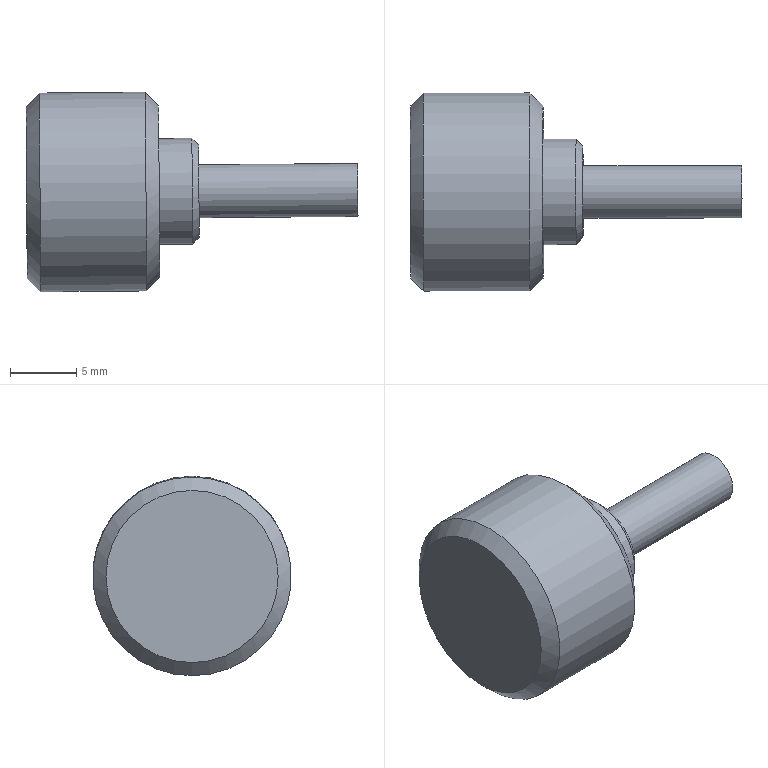Component | NX | INDICATOR_LOCK_HANDWHEEL | 1 solid | 10 faces | box 25.06 x 15.01 x 15.06 mm | volume 2021 mm3 | plane 4 | cylinder 3 | cone 3 | commonest cylinder face diameters 4 x1 8 x1 15 x1
STEP:
#1=CARTESIAN_POINT('',(0.,0.,0.));
#2=DIRECTION('',(0.,0.,1.));
#3=DIRECTION('',(1.,0.,0.));
#4=AXIS2_PLACEMENT_3D('',#1,#2,#3);
#5=CARTESIAN_POINT('',(65.216,280.465,124.861));
#6=VERTEX_POINT('',#5);
#7=CARTESIAN_POINT('',(65.167,280.465,131.36));
#8=DIRECTION('',(-1.,-0.001327,-0.007524));
#9=DIRECTION('',(0.007524,0.00000499,-1.));
#10=AXIS2_PLACEMENT_3D('',#7,#8,#9);
#11=CIRCLE('',#10,6.5);
#12=CARTESIAN_POINT('',(65.11,280.465,138.86));
#13=DIRECTION('',(1.,0.001327,0.007524));
#14=DIRECTION('',(0.007524,0.00000499,-1.));
#15=AXIS2_PLACEMENT_3D('',#12,#13,#14);
#16=PLANE('',#15);
#17=CARTESIAN_POINT('',(14.,-0.));
#18=CARTESIAN_POINT('',(14.,-11.258));
#19=CARTESIAN_POINT('',(4.25,-5.629));
#20=CARTESIAN_POINT('',(-5.5,-0.));
#21=CARTESIAN_POINT('',(4.25,5.629));
#22=CARTESIAN_POINT('',(14.,11.258));
#23=CARTESIAN_POINT('',(14.,-0.));
#24=(BOUNDED_CURVE()B_SPLINE_CURVE(2,(#17,#18,#19,#20,#21,#22,#23),.UNSPECIFIED.,.T.,.F.)B_SPLINE_CURVE_WITH_KNOTS((1,2,2,2,2,1),(-2.094,0.,2.094,4.189,6.283,8.378),.UNSPECIFIED.)CURVE()GEOMETRIC_REPRESENTATION_ITEM()RATIONAL_B_SPLINE_CURVE((1.,0.5,1.,0.5,1.,0.5,1.))REPRESENTATION_ITEM(''));
#25=(GEOMETRIC_REPRESENTATION_CONTEXT(2)PARAMETRIC_REPRESENTATION_CONTEXT()REPRESENTATION_CONTEXT('',''));
#26=DEFINITIONAL_REPRESENTATION('',(#24),#25);
#27=PCURVE('',#16,#26);
#28=CARTESIAN_POINT('',(65.167,280.465,131.36));
#29=DIRECTION('',(1.,0.001327,0.007524));
#30=DIRECTION('',(0.007524,0.00000499,-1.));
#31=AXIS2_PLACEMENT_3D('',#28,#29,#30);
#32=CONICAL_SURFACE('',#31,6.5,0.7854);
#33=CARTESIAN_POINT('',(6.283,0.));
#34=DIRECTION('',(-1.,0.));
#35=VECTOR('',#34,1.);
#36=LINE('',#33,#35);
#37=(GEOMETRIC_REPRESENTATION_CONTEXT(2)PARAMETRIC_REPRESENTATION_CONTEXT()REPRESENTATION_CONTEXT('',''));
#38=DEFINITIONAL_REPRESENTATION('',(#36),#37);
#39=PCURVE('',#32,#38);
#40=SURFACE_CURVE('',#11,(#27,#39),.PCURVE_S1.);
#41=EDGE_CURVE('',#6,#6,#40,.T.);
#42=ORIENTED_EDGE('',*,*,#41,.T.);
#43=EDGE_LOOP('',(#42));
#44=FACE_BOUND('',#43,.T.);
#45=ADVANCED_FACE('',(#44),#16,.F.);
#46=CARTESIAN_POINT('',(90.151,280.498,133.548));
#47=VERTEX_POINT('',#46);
#48=CARTESIAN_POINT('',(90.166,280.498,131.548));
#49=DIRECTION('',(-1.,-0.001327,-0.007524));
#50=DIRECTION('',(-0.007524,-0.00000499,1.));
#51=AXIS2_PLACEMENT_3D('',#48,#49,#50);
#52=CIRCLE('',#51,2.);
#53=CARTESIAN_POINT('',(90.166,280.498,131.548));
#54=DIRECTION('',(-1.,-0.001327,-0.007524));
#55=DIRECTION('',(-0.007524,-0.00000499,1.));
#56=AXIS2_PLACEMENT_3D('',#53,#54,#55);
#57=PLANE('',#56);
#58=CARTESIAN_POINT('',(0.,0.));
#59=DIRECTION('',(1.,-0.));
#60=AXIS2_PLACEMENT_2D('',#58,#59);
#61=CIRCLE('',#60,2.);
#62=(GEOMETRIC_REPRESENTATION_CONTEXT(2)PARAMETRIC_REPRESENTATION_CONTEXT()REPRESENTATION_CONTEXT('',''));
#63=DEFINITIONAL_REPRESENTATION('',(#61),#62);
#64=PCURVE('',#57,#63);
#65=CARTESIAN_POINT('',(90.166,280.498,131.548));
#66=DIRECTION('',(-1.,-0.001327,-0.007524));
#67=DIRECTION('',(-0.007524,-0.00000499,1.));
#68=AXIS2_PLACEMENT_3D('',#65,#66,#67);
#69=CYLINDRICAL_SURFACE('',#68,2.);
#70=CARTESIAN_POINT('',(0.,-0.));
#71=DIRECTION('',(1.,0.));
#72=VECTOR('',#71,1.);
#73=LINE('',#70,#72);
#74=(GEOMETRIC_REPRESENTATION_CONTEXT(2)PARAMETRIC_REPRESENTATION_CONTEXT()REPRESENTATION_CONTEXT('',''));
#75=DEFINITIONAL_REPRESENTATION('',(#73),#74);
#76=PCURVE('',#69,#75);
#77=SURFACE_CURVE('',#52,(#64,#76),.PCURVE_S1.);
#78=EDGE_CURVE('',#47,#47,#77,.T.);
#79=ORIENTED_EDGE('',*,*,#78,.F.);
#80=EDGE_LOOP('',(#79));
#81=FACE_BOUND('',#80,.T.);
#82=ADVANCED_FACE('',(#81),#57,.F.);
#83=CARTESIAN_POINT('',(78.151,280.482,133.458));
#84=VERTEX_POINT('',#83);
#85=CARTESIAN_POINT('',(78.166,280.482,131.458));
#86=DIRECTION('',(-1.,-0.001327,-0.007524));
#87=DIRECTION('',(-0.007524,-0.00000499,1.));
#88=AXIS2_PLACEMENT_3D('',#85,#86,#87);
#89=CIRCLE('',#88,2.);
#90=CARTESIAN_POINT('',(0.,12.));
#91=DIRECTION('',(1.,0.));
#92=VECTOR('',#91,1.);
#93=LINE('',#90,#92);
#94=(GEOMETRIC_REPRESENTATION_CONTEXT(2)PARAMETRIC_REPRESENTATION_CONTEXT()REPRESENTATION_CONTEXT('',''));
#95=DEFINITIONAL_REPRESENTATION('',(#93),#94);
#96=PCURVE('',#69,#95);
#97=CARTESIAN_POINT('',(78.151,280.482,133.458));
#98=DIRECTION('',(-1.,-0.001327,-0.007524));
#99=DIRECTION('',(-0.007524,-0.00000499,1.));
#100=AXIS2_PLACEMENT_3D('',#97,#98,#99);
#101=PLANE('',#100);
#102=CARTESIAN_POINT('',(-2.,0.));
#103=DIRECTION('',(1.,-0.));
#104=AXIS2_PLACEMENT_2D('',#102,#103);
#105=CIRCLE('',#104,2.);
#106=(GEOMETRIC_REPRESENTATION_CONTEXT(2)PARAMETRIC_REPRESENTATION_CONTEXT()REPRESENTATION_CONTEXT('',''));
#107=DEFINITIONAL_REPRESENTATION('',(#105),#106);
#108=PCURVE('',#101,#107);
#109=SURFACE_CURVE('',#89,(#96,#108),.PCURVE_S1.);
#110=EDGE_CURVE('',#84,#84,#109,.T.);
#111=ORIENTED_EDGE('',*,*,#110,.F.);
#112=CARTESIAN_POINT('',(90.151,280.498,133.548));
#113=CARTESIAN_POINT('',(78.151,280.482,133.458));
#114=B_SPLINE_CURVE_WITH_KNOTS('',1,(#112,#113),.UNSPECIFIED.,.F.,.F.,(2,2),(-0.,12.),.PIECEWISE_BEZIER_KNOTS.);
#115=CARTESIAN_POINT('',(0.,0.));
#116=DIRECTION('',(0.,1.));
#117=VECTOR('',#116,1.);
#118=LINE('',#115,#117);
#119=(GEOMETRIC_REPRESENTATION_CONTEXT(2)PARAMETRIC_REPRESENTATION_CONTEXT()REPRESENTATION_CONTEXT('',''));
#120=DEFINITIONAL_REPRESENTATION('',(#118),#119);
#121=PCURVE('',#69,#120);
#122=CARTESIAN_POINT('',(6.283,0.));
#123=DIRECTION('',(0.,1.));
#124=VECTOR('',#123,1.);
#125=LINE('',#122,#124);
#126=(GEOMETRIC_REPRESENTATION_CONTEXT(2)PARAMETRIC_REPRESENTATION_CONTEXT()REPRESENTATION_CONTEXT('',''));
#127=DEFINITIONAL_REPRESENTATION('',(#125),#126);
#128=PCURVE('',#69,#127);
#129=SEAM_CURVE('',#114,(#121,#128),.PCURVE_S1.);
#130=EDGE_CURVE('',#47,#84,#129,.T.);
#131=ORIENTED_EDGE('',*,*,#130,.F.);
#132=ORIENTED_EDGE('',*,*,#78,.T.);
#133=ORIENTED_EDGE('',*,*,#130,.T.);
#134=EDGE_LOOP('',(#111,#131,#132,#133));
#135=FACE_BOUND('',#134,.T.);
#136=ADVANCED_FACE('',(#135),#69,.T.);
#137=CARTESIAN_POINT('',(78.14,280.482,134.958));
#138=VERTEX_POINT('',#137);
#139=CARTESIAN_POINT('',(78.166,280.482,131.458));
#140=DIRECTION('',(1.,0.001327,0.007524));
#141=DIRECTION('',(-0.007524,-0.00000499,1.));
#142=AXIS2_PLACEMENT_3D('',#139,#140,#141);
#143=CIRCLE('',#142,3.5);
#144=CARTESIAN_POINT('',(1.5,0.));
#145=CARTESIAN_POINT('',(1.5,-6.062));
#146=CARTESIAN_POINT('',(-3.75,-3.031));
#147=CARTESIAN_POINT('',(-9.,0.));
#148=CARTESIAN_POINT('',(-3.75,3.031));
#149=CARTESIAN_POINT('',(1.5,6.062));
#150=CARTESIAN_POINT('',(1.5,0.));
#151=(BOUNDED_CURVE()B_SPLINE_CURVE(2,(#144,#145,#146,#147,#148,#149,#150),.UNSPECIFIED.,.T.,.F.)B_SPLINE_CURVE_WITH_KNOTS((1,2,2,2,2,1),(-2.094,0.,2.094,4.189,6.283,8.378),.UNSPECIFIED.)CURVE()GEOMETRIC_REPRESENTATION_ITEM()RATIONAL_B_SPLINE_CURVE((1.,0.5,1.,0.5,1.,0.5,1.))REPRESENTATION_ITEM(''));
#152=(GEOMETRIC_REPRESENTATION_CONTEXT(2)PARAMETRIC_REPRESENTATION_CONTEXT()REPRESENTATION_CONTEXT('',''));
#153=DEFINITIONAL_REPRESENTATION('',(#151),#152);
#154=PCURVE('',#101,#153);
#155=CARTESIAN_POINT('',(77.666,280.481,131.454));
#156=DIRECTION('',(-1.,-0.001327,-0.007524));
#157=DIRECTION('',(-0.007524,-0.00000499,1.));
#158=AXIS2_PLACEMENT_3D('',#155,#156,#157);
#159=CONICAL_SURFACE('',#158,4.,0.7854);
#160=CARTESIAN_POINT('',(6.283,-0.5));
#161=DIRECTION('',(-1.,0.));
#162=VECTOR('',#161,1.);
#163=LINE('',#160,#162);
#164=(GEOMETRIC_REPRESENTATION_CONTEXT(2)PARAMETRIC_REPRESENTATION_CONTEXT()REPRESENTATION_CONTEXT('',''));
#165=DEFINITIONAL_REPRESENTATION('',(#163),#164);
#166=PCURVE('',#159,#165);
#167=SURFACE_CURVE('',#143,(#154,#166),.PCURVE_S1.);
#168=EDGE_CURVE('',#138,#138,#167,.T.);
#169=ORIENTED_EDGE('',*,*,#168,.T.);
#170=EDGE_LOOP('',(#169));
#171=FACE_BOUND('',#170,.T.);
#172=ORIENTED_EDGE('',*,*,#110,.T.);
#173=EDGE_LOOP('',(#172));
#174=FACE_BOUND('',#173,.T.);
#175=ADVANCED_FACE('',(#171,#174),#101,.F.);
#176=CARTESIAN_POINT('',(77.636,280.481,135.454));
#177=VERTEX_POINT('',#176);
#178=CARTESIAN_POINT('',(77.666,280.481,131.454));
#179=DIRECTION('',(-1.,-0.001327,-0.007524));
#180=DIRECTION('',(-0.007524,-0.00000499,1.));
#181=AXIS2_PLACEMENT_3D('',#178,#179,#180);
#182=CIRCLE('',#181,4.);
#183=CARTESIAN_POINT('',(90.166,280.498,131.548));
#184=DIRECTION('',(-1.,-0.001327,-0.007524));
#185=DIRECTION('',(-0.007524,-0.00000499,1.));
#186=AXIS2_PLACEMENT_3D('',#183,#184,#185);
#187=CYLINDRICAL_SURFACE('',#186,4.);
#188=CARTESIAN_POINT('',(0.,12.5));
#189=DIRECTION('',(1.,0.));
#190=VECTOR('',#189,1.);
#191=LINE('',#188,#190);
#192=(GEOMETRIC_REPRESENTATION_CONTEXT(2)PARAMETRIC_REPRESENTATION_CONTEXT()REPRESENTATION_CONTEXT('',''));
#193=DEFINITIONAL_REPRESENTATION('',(#191),#192);
#194=PCURVE('',#187,#193);
#195=CARTESIAN_POINT('',(0.,-0.));
#196=DIRECTION('',(1.,0.));
#197=VECTOR('',#196,1.);
#198=LINE('',#195,#197);
#199=(GEOMETRIC_REPRESENTATION_CONTEXT(2)PARAMETRIC_REPRESENTATION_CONTEXT()REPRESENTATION_CONTEXT('',''));
#200=DEFINITIONAL_REPRESENTATION('',(#198),#199);
#201=PCURVE('',#159,#200);
#202=SURFACE_CURVE('',#182,(#194,#201),.PCURVE_S1.);
#203=EDGE_CURVE('',#177,#177,#202,.T.);
#204=ORIENTED_EDGE('',*,*,#203,.T.);
#205=CARTESIAN_POINT('',(75.136,280.478,135.435));
#206=VERTEX_POINT('',#205);
#207=CARTESIAN_POINT('',(77.636,280.481,135.454));
#208=CARTESIAN_POINT('',(75.136,280.478,135.435));
#209=B_SPLINE_CURVE_WITH_KNOTS('',1,(#207,#208),.UNSPECIFIED.,.F.,.F.,(2,2),(12.5,15.),.PIECEWISE_BEZIER_KNOTS.);
#210=CARTESIAN_POINT('',(6.283,0.));
#211=DIRECTION('',(0.,1.));
#212=VECTOR('',#211,1.);
#213=LINE('',#210,#212);
#214=(GEOMETRIC_REPRESENTATION_CONTEXT(2)PARAMETRIC_REPRESENTATION_CONTEXT()REPRESENTATION_CONTEXT('',''));
#215=DEFINITIONAL_REPRESENTATION('',(#213),#214);
#216=PCURVE('',#187,#215);
#217=CARTESIAN_POINT('',(0.,0.));
#218=DIRECTION('',(0.,1.));
#219=VECTOR('',#218,1.);
#220=LINE('',#217,#219);
#221=(GEOMETRIC_REPRESENTATION_CONTEXT(2)PARAMETRIC_REPRESENTATION_CONTEXT()REPRESENTATION_CONTEXT('',''));
#222=DEFINITIONAL_REPRESENTATION('',(#220),#221);
#223=PCURVE('',#187,#222);
#224=SEAM_CURVE('',#209,(#216,#223),.PCURVE_S1.);
#225=EDGE_CURVE('',#177,#206,#224,.T.);
#226=ORIENTED_EDGE('',*,*,#225,.T.);
#227=CARTESIAN_POINT('',(75.166,280.478,131.436));
#228=DIRECTION('',(-1.,-0.001327,-0.007524));
#229=DIRECTION('',(-0.007524,-0.00000499,1.));
#230=AXIS2_PLACEMENT_3D('',#227,#228,#229);
#231=CIRCLE('',#230,4.);
#232=CARTESIAN_POINT('',(0.,15.));
#233=DIRECTION('',(1.,0.));
#234=VECTOR('',#233,1.);
#235=LINE('',#232,#234);
#236=(GEOMETRIC_REPRESENTATION_CONTEXT(2)PARAMETRIC_REPRESENTATION_CONTEXT()REPRESENTATION_CONTEXT('',''));
#237=DEFINITIONAL_REPRESENTATION('',(#235),#236);
#238=PCURVE('',#187,#237);
#239=CARTESIAN_POINT('',(75.136,280.478,135.435));
#240=DIRECTION('',(-1.,-0.001327,-0.007524));
#241=DIRECTION('',(-0.007524,-0.00000499,1.));
#242=AXIS2_PLACEMENT_3D('',#239,#240,#241);
#243=PLANE('',#242);
#244=CARTESIAN_POINT('',(-4.,-0.));
#245=DIRECTION('',(1.,-0.));
#246=AXIS2_PLACEMENT_2D('',#244,#245);
#247=CIRCLE('',#246,4.);
#248=(GEOMETRIC_REPRESENTATION_CONTEXT(2)PARAMETRIC_REPRESENTATION_CONTEXT()REPRESENTATION_CONTEXT('',''));
#249=DEFINITIONAL_REPRESENTATION('',(#247),#248);
#250=PCURVE('',#243,#249);
#251=SURFACE_CURVE('',#231,(#238,#250),.PCURVE_S1.);
#252=EDGE_CURVE('',#206,#206,#251,.T.);
#253=ORIENTED_EDGE('',*,*,#252,.F.);
#254=ORIENTED_EDGE('',*,*,#225,.F.);
#255=EDGE_LOOP('',(#204,#226,#253,#254));
#256=FACE_BOUND('',#255,.T.);
#257=ADVANCED_FACE('',(#256),#187,.T.);
#258=CARTESIAN_POINT('',(75.118,280.478,137.935));
#259=VERTEX_POINT('',#258);
#260=CARTESIAN_POINT('',(75.166,280.478,131.436));
#261=DIRECTION('',(1.,0.001327,0.007524));
#262=DIRECTION('',(-0.007524,-0.00000499,1.));
#263=AXIS2_PLACEMENT_3D('',#260,#261,#262);
#264=CIRCLE('',#263,6.5);
#265=CARTESIAN_POINT('',(2.5,-0.));
#266=CARTESIAN_POINT('',(2.5,-11.258));
#267=CARTESIAN_POINT('',(-7.25,-5.629));
#268=CARTESIAN_POINT('',(-17.,-0.));
#269=CARTESIAN_POINT('',(-7.25,5.629));
#270=CARTESIAN_POINT('',(2.5,11.258));
#271=CARTESIAN_POINT('',(2.5,-0.));
#272=(BOUNDED_CURVE()B_SPLINE_CURVE(2,(#265,#266,#267,#268,#269,#270,#271),.UNSPECIFIED.,.T.,.F.)B_SPLINE_CURVE_WITH_KNOTS((1,2,2,2,2,1),(-2.094,0.,2.094,4.189,6.283,8.378),.UNSPECIFIED.)CURVE()GEOMETRIC_REPRESENTATION_ITEM()RATIONAL_B_SPLINE_CURVE((1.,0.5,1.,0.5,1.,0.5,1.))REPRESENTATION_ITEM(''));
#273=(GEOMETRIC_REPRESENTATION_CONTEXT(2)PARAMETRIC_REPRESENTATION_CONTEXT()REPRESENTATION_CONTEXT('',''));
#274=DEFINITIONAL_REPRESENTATION('',(#272),#273);
#275=PCURVE('',#243,#274);
#276=CARTESIAN_POINT('',(74.166,280.476,131.428));
#277=DIRECTION('',(-1.,-0.001327,-0.007524));
#278=DIRECTION('',(-0.007524,-0.00000499,1.));
#279=AXIS2_PLACEMENT_3D('',#276,#277,#278);
#280=CONICAL_SURFACE('',#279,7.5,0.7854);
#281=CARTESIAN_POINT('',(6.283,-1.));
#282=DIRECTION('',(-1.,0.));
#283=VECTOR('',#282,1.);
#284=LINE('',#281,#283);
#285=(GEOMETRIC_REPRESENTATION_CONTEXT(2)PARAMETRIC_REPRESENTATION_CONTEXT()REPRESENTATION_CONTEXT('',''));
#286=DEFINITIONAL_REPRESENTATION('',(#284),#285);
#287=PCURVE('',#280,#286);
#288=SURFACE_CURVE('',#264,(#275,#287),.PCURVE_S1.);
#289=EDGE_CURVE('',#259,#259,#288,.T.);
#290=ORIENTED_EDGE('',*,*,#289,.T.);
#291=EDGE_LOOP('',(#290));
#292=FACE_BOUND('',#291,.T.);
#293=ORIENTED_EDGE('',*,*,#252,.T.);
#294=EDGE_LOOP('',(#293));
#295=FACE_BOUND('',#294,.T.);
#296=ADVANCED_FACE('',(#292,#295),#243,.F.);
#297=CARTESIAN_POINT('',(66.223,280.466,123.868));
#298=VERTEX_POINT('',#297);
#299=CARTESIAN_POINT('',(66.11,280.466,138.868));
#300=VERTEX_POINT('',#299);
#301=CARTESIAN_POINT('',(66.167,280.466,131.368));
#302=DIRECTION('',(1.,0.001327,0.007524));
#303=DIRECTION('',(0.007524,0.00000499,-1.));
#304=AXIS2_PLACEMENT_3D('',#301,#302,#303);
#305=CIRCLE('',#304,7.5);
#306=CARTESIAN_POINT('',(90.166,280.498,131.548));
#307=DIRECTION('',(-1.,-0.001327,-0.007524));
#308=DIRECTION('',(-0.007524,-0.00000499,1.));
#309=AXIS2_PLACEMENT_3D('',#306,#307,#308);
#310=CYLINDRICAL_SURFACE('',#309,7.5);
#311=CARTESIAN_POINT('',(3.142,24.));
#312=DIRECTION('',(-1.,0.));
#313=VECTOR('',#312,1.);
#314=LINE('',#311,#313);
#315=(GEOMETRIC_REPRESENTATION_CONTEXT(2)PARAMETRIC_REPRESENTATION_CONTEXT()REPRESENTATION_CONTEXT('',''));
#316=DEFINITIONAL_REPRESENTATION('',(#314),#315);
#317=PCURVE('',#310,#316);
#318=CARTESIAN_POINT('',(0.,1.));
#319=DIRECTION('',(1.,0.));
#320=VECTOR('',#319,1.);
#321=LINE('',#318,#320);
#322=(GEOMETRIC_REPRESENTATION_CONTEXT(2)PARAMETRIC_REPRESENTATION_CONTEXT()REPRESENTATION_CONTEXT('',''));
#323=DEFINITIONAL_REPRESENTATION('',(#321),#322);
#324=PCURVE('',#32,#323);
#325=SURFACE_CURVE('',#305,(#317,#324),.PCURVE_S1.);
#326=EDGE_CURVE('',#298,#300,#325,.T.);
#327=ORIENTED_EDGE('',*,*,#326,.T.);
#328=CARTESIAN_POINT('',(74.11,280.476,138.928));
#329=VERTEX_POINT('',#328);
#330=CARTESIAN_POINT('',(74.11,280.476,138.928));
#331=CARTESIAN_POINT('',(66.11,280.466,138.868));
#332=B_SPLINE_CURVE_WITH_KNOTS('',1,(#330,#331),.UNSPECIFIED.,.F.,.F.,(2,2),(16.,24.),.PIECEWISE_BEZIER_KNOTS.);
#333=CARTESIAN_POINT('',(0.,0.));
#334=DIRECTION('',(0.,1.));
#335=VECTOR('',#334,1.);
#336=LINE('',#333,#335);
#337=(GEOMETRIC_REPRESENTATION_CONTEXT(2)PARAMETRIC_REPRESENTATION_CONTEXT()REPRESENTATION_CONTEXT('',''));
#338=DEFINITIONAL_REPRESENTATION('',(#336),#337);
#339=PCURVE('',#310,#338);
#340=CARTESIAN_POINT('',(6.283,0.));
#341=DIRECTION('',(0.,1.));
#342=VECTOR('',#341,1.);
#343=LINE('',#340,#342);
#344=(GEOMETRIC_REPRESENTATION_CONTEXT(2)PARAMETRIC_REPRESENTATION_CONTEXT()REPRESENTATION_CONTEXT('',''));
#345=DEFINITIONAL_REPRESENTATION('',(#343),#344);
#346=PCURVE('',#310,#345);
#347=SEAM_CURVE('',#332,(#339,#346),.PCURVE_S1.);
#348=EDGE_CURVE('',#329,#300,#347,.T.);
#349=ORIENTED_EDGE('',*,*,#348,.F.);
#350=CARTESIAN_POINT('',(74.166,280.476,131.428));
#351=DIRECTION('',(-1.,-0.001327,-0.007524));
#352=DIRECTION('',(-0.007524,-0.00000499,1.));
#353=AXIS2_PLACEMENT_3D('',#350,#351,#352);
#354=CIRCLE('',#353,7.5);
#355=CARTESIAN_POINT('',(0.,16.));
#356=DIRECTION('',(1.,0.));
#357=VECTOR('',#356,1.);
#358=LINE('',#355,#357);
#359=(GEOMETRIC_REPRESENTATION_CONTEXT(2)PARAMETRIC_REPRESENTATION_CONTEXT()REPRESENTATION_CONTEXT('',''));
#360=DEFINITIONAL_REPRESENTATION('',(#358),#359);
#361=PCURVE('',#310,#360);
#362=CARTESIAN_POINT('',(0.,0.));
#363=DIRECTION('',(1.,0.));
#364=VECTOR('',#363,1.);
#365=LINE('',#362,#364);
#366=(GEOMETRIC_REPRESENTATION_CONTEXT(2)PARAMETRIC_REPRESENTATION_CONTEXT()REPRESENTATION_CONTEXT('',''));
#367=DEFINITIONAL_REPRESENTATION('',(#365),#366);
#368=PCURVE('',#280,#367);
#369=SURFACE_CURVE('',#354,(#361,#368),.PCURVE_S1.);
#370=EDGE_CURVE('',#329,#329,#369,.T.);
#371=ORIENTED_EDGE('',*,*,#370,.T.);
#372=ORIENTED_EDGE('',*,*,#348,.T.);
#373=CARTESIAN_POINT('',(66.167,280.466,131.368));
#374=DIRECTION('',(1.,0.001327,0.007524));
#375=DIRECTION('',(0.007524,0.00000499,-1.));
#376=AXIS2_PLACEMENT_3D('',#373,#374,#375);
#377=CIRCLE('',#376,7.5);
#378=CARTESIAN_POINT('',(9.425,24.));
#379=DIRECTION('',(-1.,0.));
#380=VECTOR('',#379,1.);
#381=LINE('',#378,#380);
#382=(GEOMETRIC_REPRESENTATION_CONTEXT(2)PARAMETRIC_REPRESENTATION_CONTEXT()REPRESENTATION_CONTEXT('',''));
#383=DEFINITIONAL_REPRESENTATION('',(#381),#382);
#384=PCURVE('',#310,#383);
#385=CARTESIAN_POINT('',(-0.,1.));
#386=DIRECTION('',(1.,-0.));
#387=VECTOR('',#386,1.);
#388=LINE('',#385,#387);
#389=(GEOMETRIC_REPRESENTATION_CONTEXT(2)PARAMETRIC_REPRESENTATION_CONTEXT()REPRESENTATION_CONTEXT('',''));
#390=DEFINITIONAL_REPRESENTATION('',(#388),#389);
#391=PCURVE('',#32,#390);
#392=SURFACE_CURVE('',#377,(#384,#391),.PCURVE_S1.);
#393=EDGE_CURVE('',#300,#298,#392,.T.);
#394=ORIENTED_EDGE('',*,*,#393,.T.);
#395=EDGE_LOOP('',(#327,#349,#371,#372,#394));
#396=FACE_BOUND('',#395,.T.);
#397=ADVANCED_FACE('',(#396),#310,.T.);
#398=ORIENTED_EDGE('',*,*,#326,.F.);
#399=CARTESIAN_POINT('',(65.216,280.465,124.861));
#400=CARTESIAN_POINT('',(66.223,280.466,123.868));
#401=B_SPLINE_CURVE_WITH_KNOTS('',1,(#399,#400),.UNSPECIFIED.,.F.,.F.,(2,2),(0.,1.414),.PIECEWISE_BEZIER_KNOTS.);
#402=CARTESIAN_POINT('',(0.,0.));
#403=DIRECTION('',(0.,1.));
#404=VECTOR('',#403,1.);
#405=LINE('',#402,#404);
#406=(GEOMETRIC_REPRESENTATION_CONTEXT(2)PARAMETRIC_REPRESENTATION_CONTEXT()REPRESENTATION_CONTEXT('',''));
#407=DEFINITIONAL_REPRESENTATION('',(#405),#406);
#408=PCURVE('',#32,#407);
#409=CARTESIAN_POINT('',(6.283,0.));
#410=DIRECTION('',(0.,1.));
#411=VECTOR('',#410,1.);
#412=LINE('',#409,#411);
#413=(GEOMETRIC_REPRESENTATION_CONTEXT(2)PARAMETRIC_REPRESENTATION_CONTEXT()REPRESENTATION_CONTEXT('',''));
#414=DEFINITIONAL_REPRESENTATION('',(#412),#413);
#415=PCURVE('',#32,#414);
#416=SEAM_CURVE('',#401,(#408,#415),.PCURVE_S1.);
#417=EDGE_CURVE('',#6,#298,#416,.T.);
#418=ORIENTED_EDGE('',*,*,#417,.F.);
#419=ORIENTED_EDGE('',*,*,#41,.F.);
#420=ORIENTED_EDGE('',*,*,#417,.T.);
#421=ORIENTED_EDGE('',*,*,#393,.F.);
#422=EDGE_LOOP('',(#398,#418,#419,#420,#421));
#423=FACE_BOUND('',#422,.T.);
#424=ADVANCED_FACE('',(#423),#32,.T.);
#425=ORIENTED_EDGE('',*,*,#289,.F.);
#426=CARTESIAN_POINT('',(75.118,280.478,137.935));
#427=CARTESIAN_POINT('',(74.11,280.476,138.928));
#428=B_SPLINE_CURVE_WITH_KNOTS('',1,(#426,#427),.UNSPECIFIED.,.F.,.F.,(2,2),(-1.414,0.),.PIECEWISE_BEZIER_KNOTS.);
#429=CARTESIAN_POINT('',(6.283,0.));
#430=DIRECTION('',(0.,1.));
#431=VECTOR('',#430,1.);
#432=LINE('',#429,#431);
#433=(GEOMETRIC_REPRESENTATION_CONTEXT(2)PARAMETRIC_REPRESENTATION_CONTEXT()REPRESENTATION_CONTEXT('',''));
#434=DEFINITIONAL_REPRESENTATION('',(#432),#433);
#435=PCURVE('',#280,#434);
#436=CARTESIAN_POINT('',(0.,0.));
#437=DIRECTION('',(0.,1.));
#438=VECTOR('',#437,1.);
#439=LINE('',#436,#438);
#440=(GEOMETRIC_REPRESENTATION_CONTEXT(2)PARAMETRIC_REPRESENTATION_CONTEXT()REPRESENTATION_CONTEXT('',''));
#441=DEFINITIONAL_REPRESENTATION('',(#439),#440);
#442=PCURVE('',#280,#441);
#443=SEAM_CURVE('',#428,(#435,#442),.PCURVE_S1.);
#444=EDGE_CURVE('',#259,#329,#443,.T.);
#445=ORIENTED_EDGE('',*,*,#444,.T.);
#446=ORIENTED_EDGE('',*,*,#370,.F.);
#447=ORIENTED_EDGE('',*,*,#444,.F.);
#448=EDGE_LOOP('',(#425,#445,#446,#447));
#449=FACE_BOUND('',#448,.T.);
#450=ADVANCED_FACE('',(#449),#280,.T.);
#451=ORIENTED_EDGE('',*,*,#168,.F.);
#452=CARTESIAN_POINT('',(78.14,280.482,134.958));
#453=CARTESIAN_POINT('',(77.636,280.481,135.454));
#454=B_SPLINE_CURVE_WITH_KNOTS('',1,(#452,#453),.UNSPECIFIED.,.F.,.F.,(2,2),(-0.7071,-0.),.PIECEWISE_BEZIER_KNOTS.);
#455=CARTESIAN_POINT('',(6.283,0.));
#456=DIRECTION('',(0.,1.));
#457=VECTOR('',#456,1.);
#458=LINE('',#455,#457);
#459=(GEOMETRIC_REPRESENTATION_CONTEXT(2)PARAMETRIC_REPRESENTATION_CONTEXT()REPRESENTATION_CONTEXT('',''));
#460=DEFINITIONAL_REPRESENTATION('',(#458),#459);
#461=PCURVE('',#159,#460);
#462=CARTESIAN_POINT('',(0.,0.));
#463=DIRECTION('',(0.,1.));
#464=VECTOR('',#463,1.);
#465=LINE('',#462,#464);
#466=(GEOMETRIC_REPRESENTATION_CONTEXT(2)PARAMETRIC_REPRESENTATION_CONTEXT()REPRESENTATION_CONTEXT('',''));
#467=DEFINITIONAL_REPRESENTATION('',(#465),#466);
#468=PCURVE('',#159,#467);
#469=SEAM_CURVE('',#454,(#461,#468),.PCURVE_S1.);
#470=EDGE_CURVE('',#138,#177,#469,.T.);
#471=ORIENTED_EDGE('',*,*,#470,.T.);
#472=ORIENTED_EDGE('',*,*,#203,.F.);
#473=ORIENTED_EDGE('',*,*,#470,.F.);
#474=EDGE_LOOP('',(#451,#471,#472,#473));
#475=FACE_BOUND('',#474,.T.);
#476=ADVANCED_FACE('',(#475),#159,.T.);
#477=CLOSED_SHELL('',(#45,#82,#136,#175,#257,#296,#397,#424,#450,#476));
#478=MANIFOLD_SOLID_BREP('',#477);
#479=(LENGTH_UNIT()NAMED_UNIT(*)SI_UNIT(.MILLI.,.METRE.));
#480=UNCERTAINTY_MEASURE_WITH_UNIT(LENGTH_MEASURE(0.00001),#479,'','');
#481=(NAMED_UNIT(*)PLANE_ANGLE_UNIT()SI_UNIT($,.RADIAN.));
#482=(NAMED_UNIT(*)SI_UNIT($,.STERADIAN.)SOLID_ANGLE_UNIT());
#483=(GEOMETRIC_REPRESENTATION_CONTEXT(3)GLOBAL_UNCERTAINTY_ASSIGNED_CONTEXT((#480))GLOBAL_UNIT_ASSIGNED_CONTEXT((#479,#481,#482))REPRESENTATION_CONTEXT('',''));
#484=ADVANCED_BREP_SHAPE_REPRESENTATION('',(#4,#478),#483);